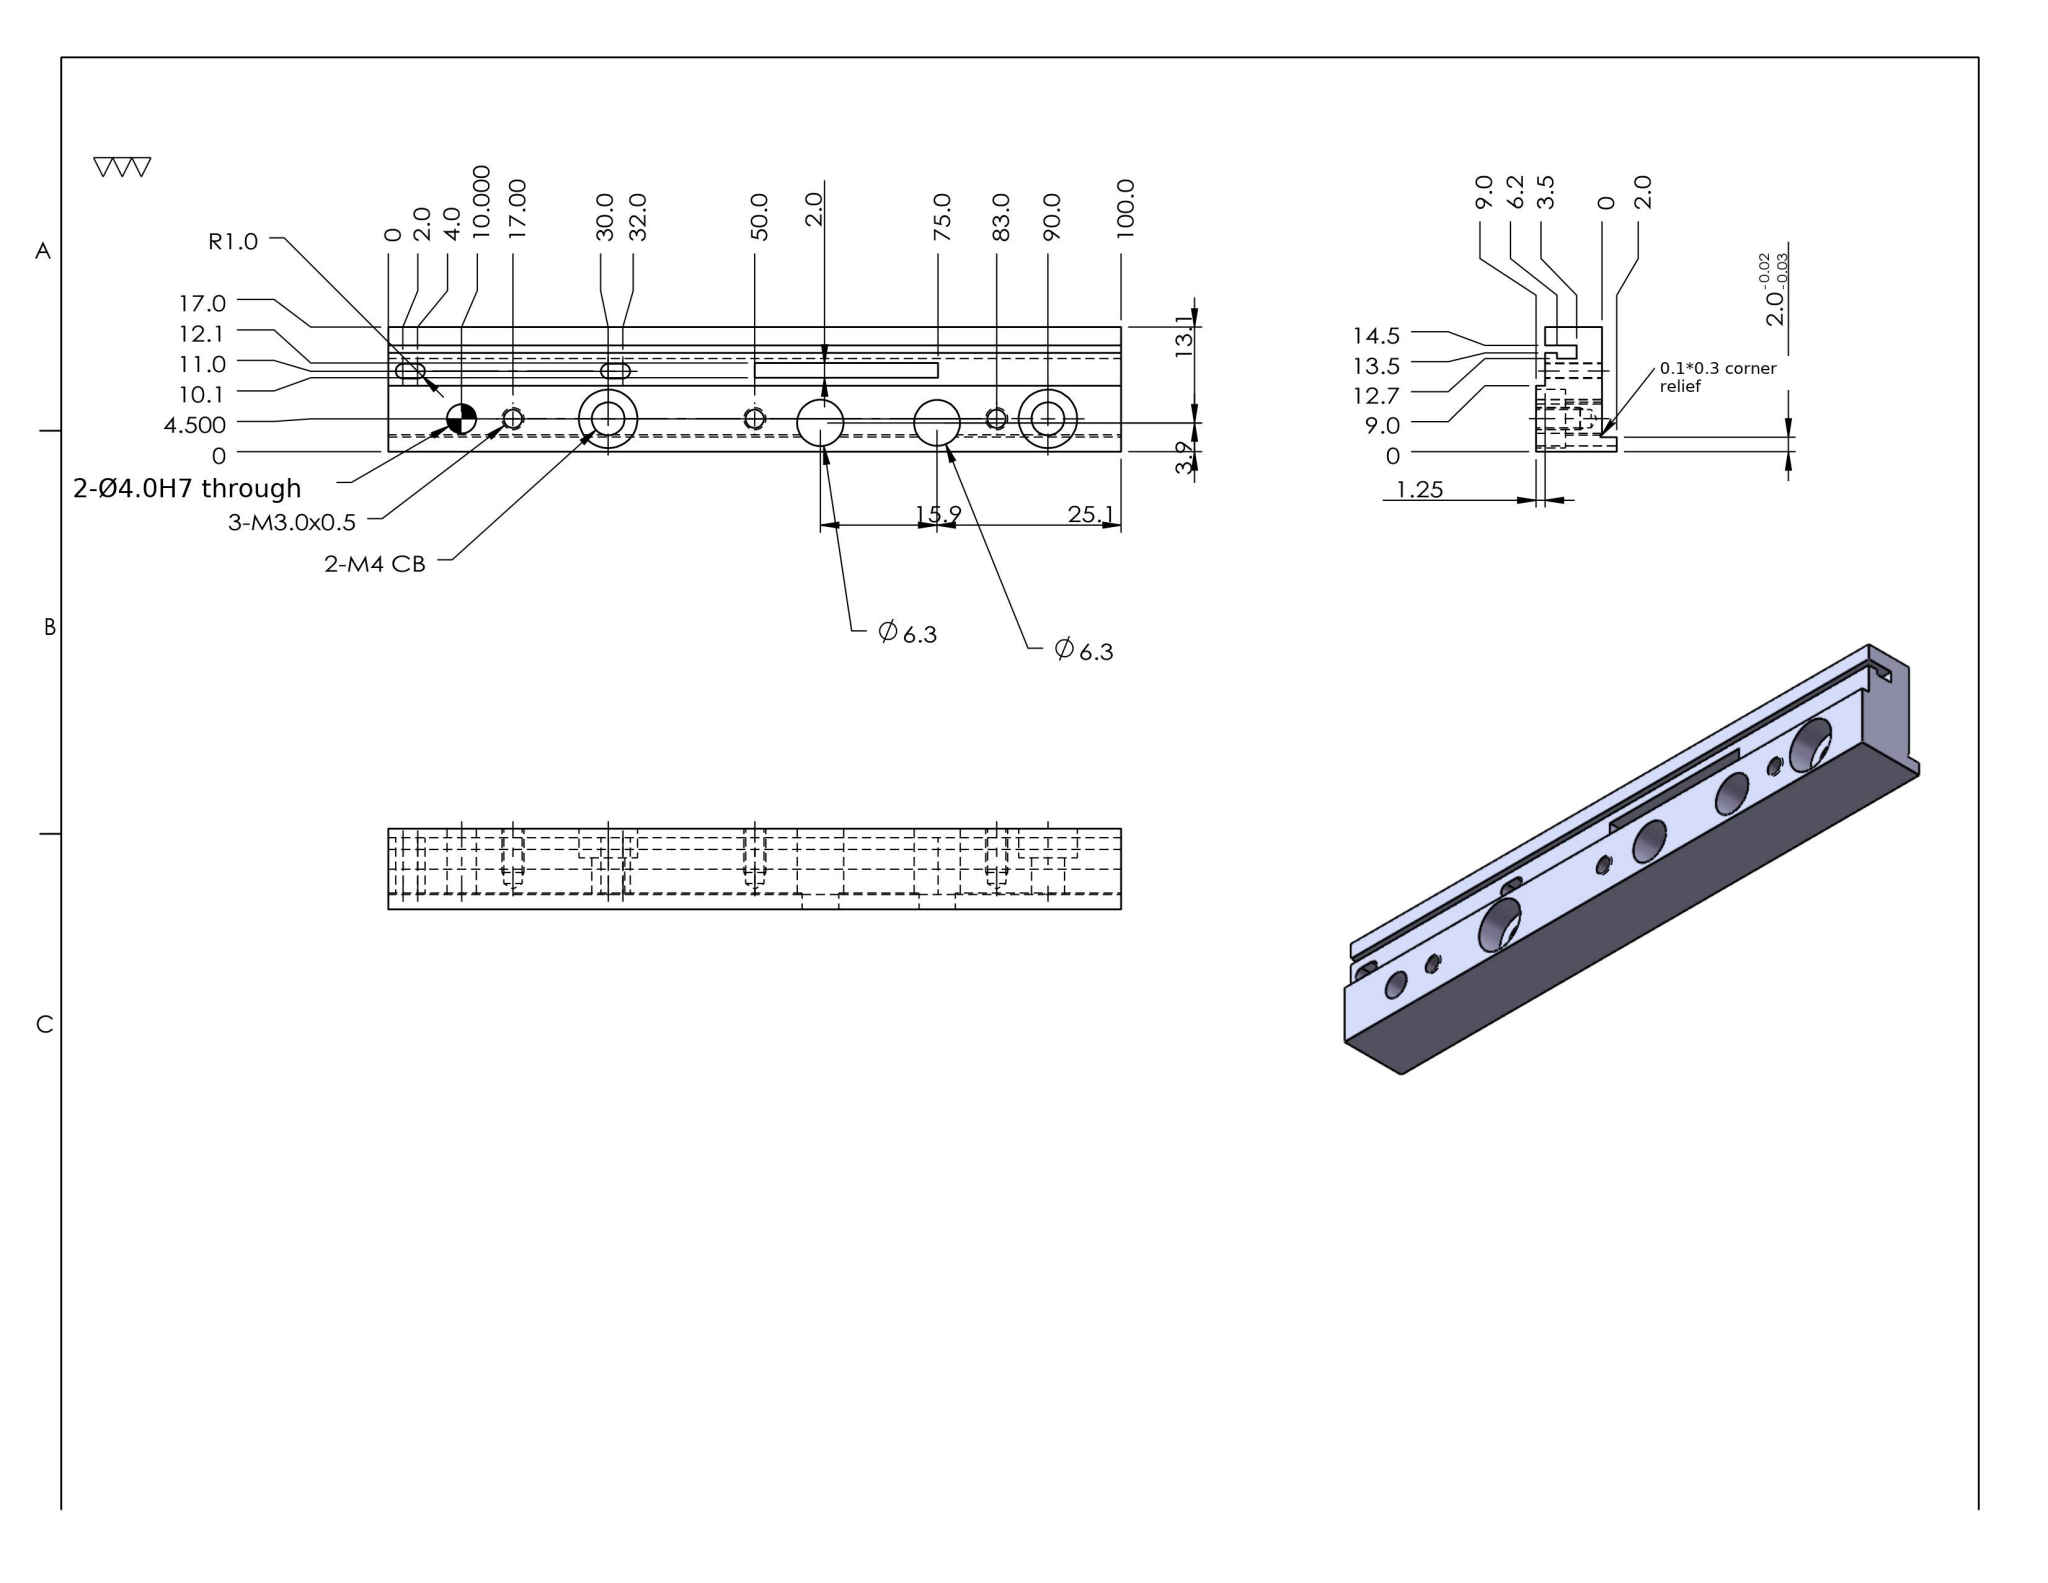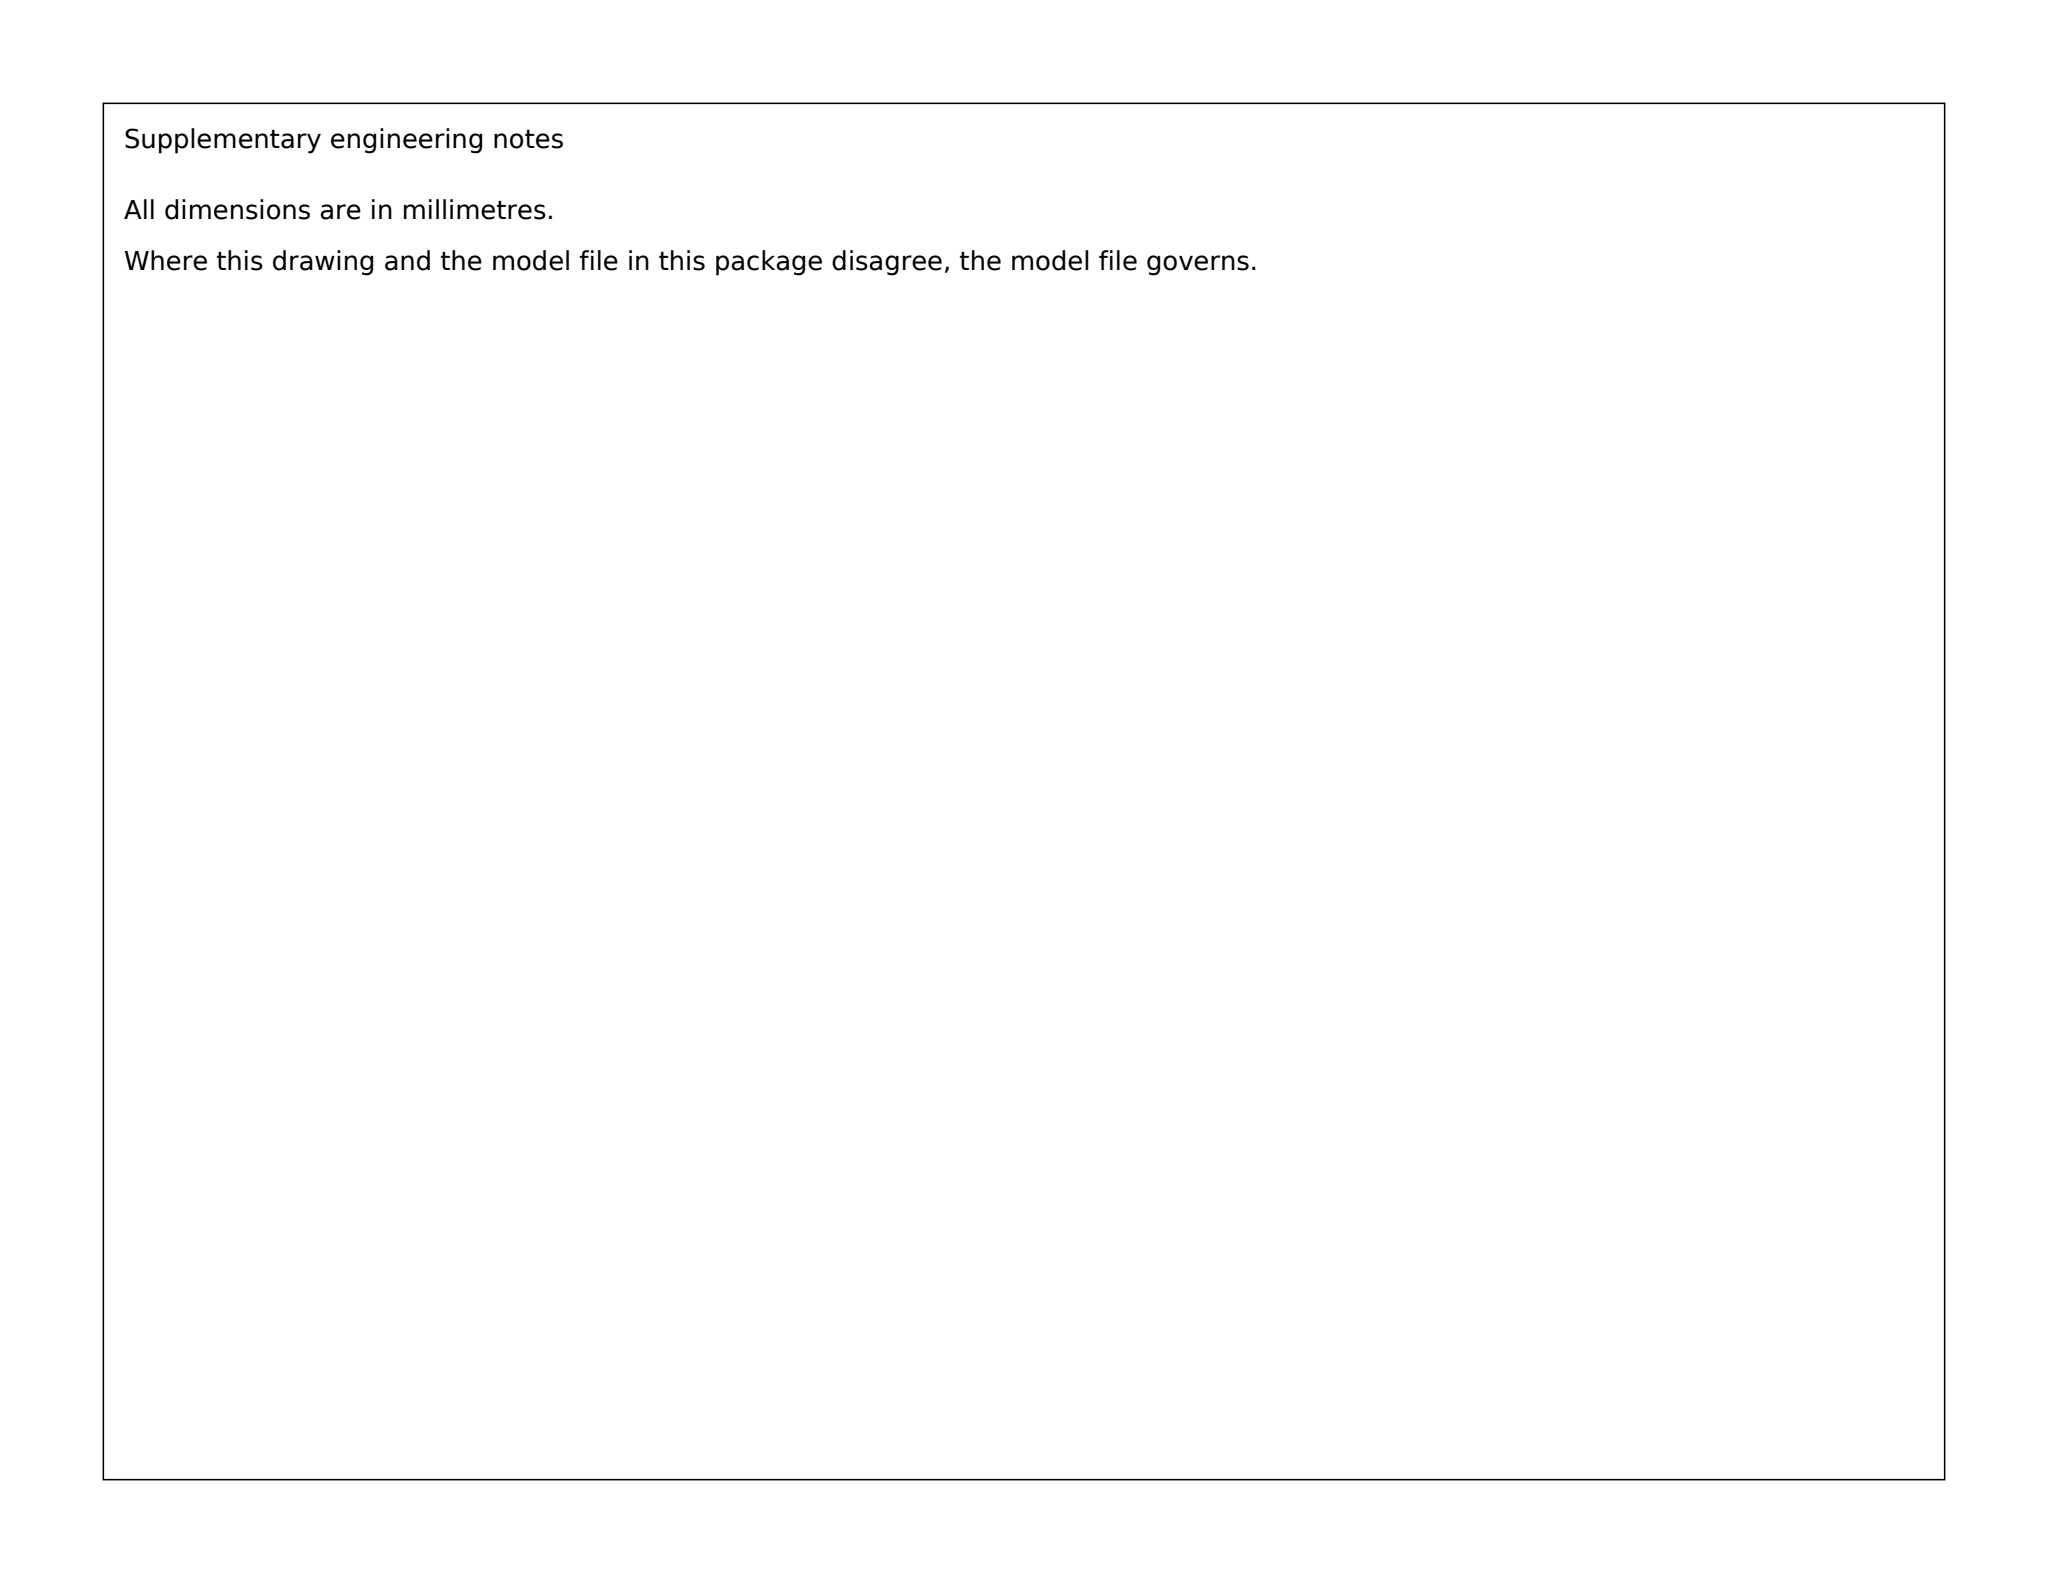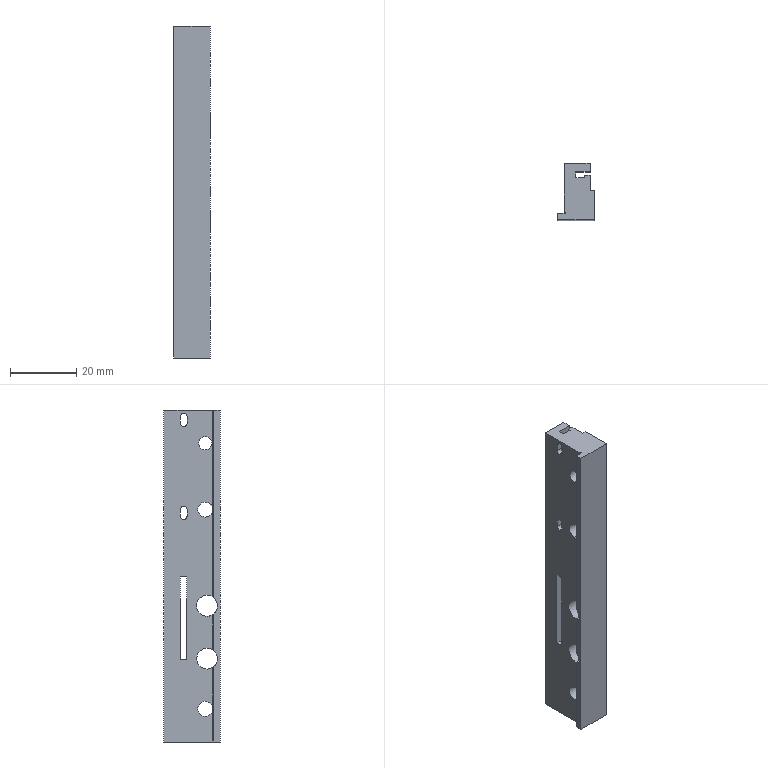Part | SolidWorks | mm | 1 solid | 68 faces | box 11 x 17 x 100 mm | volume 12182 mm3 | plane 36 | cylinder 26 | cone 6 | commonest cylinder face diameters 2.5 x6 2 x6 8 x4 4.5 x4 6.339 x2 6.289 x2 4 x2
build123d program:
from build123d import *

# Parameters (mm, degrees)
SKETCH1_W                                            = 240
SKETCH1_H                                            = 30
EXTRUDE1_DEPTH                                       = 9
SKETCH2_W                                            = 240
SKETCH2_H                                            = 8
EXTRUDE2_DEPTH                                       = 1.25
SKETCH3_W                                            = 4.3
SKETCH3_H                                            = 1
EXTRUDE3_DEPTH                                       = 243.035
SKETCH5_W                                            = 9
SKETCH5_H                                            = 9
CUT_EXTRUDE1_DEPTH                                   = 243.035
CHAMFER1_SIZE                                        = 0.5
CHAMFER1_SIZE2                                       = 3
CHAMFER2_SIZE                                        = 3
CHAMFER2_SIZE2                                       = 0.5
CHAMFER3_SIZE                                        = 0.3
CHAMFER3_SIZE2                                       = 3
CYLINDRICAL_COUNTERSUNK_HOLE_FOR_M4_SOCK_D           = 4.5
CYLINDRICAL_COUNTERSUNK_HOLE_FOR_M4_SOCK_CBORE_D     = 8
CYLINDRICAL_COUNTERSUNK_HOLE_FOR_M4_SOCK_CBORE_DEPTH = 4
LPATTERN1_COUNT                                      = 4
LPATTERN1_PITCH                                      = 60
SKETCH8_W                                            = 2
SKETCH8_H                                            = 2
EXTRUDE5_DEPTH                                       = 240
SKETCH9_W                                            = 0.2
SKETCH9_H                                            = 0.3
EXTRUDE6_DEPTH                                       = 242.085
SKETCH10_W                                           = 9
SKETCH10_H                                           = 4
EXTRUDE7_DEPTH                                       = 242.085
SKETCH11_R                                           = 2
CUT_EXTRUDE2_DEPTH                                   = 241.853
SKETCH12_W                                           = 2.7
SKETCH12_H                                           = 0.8
EXTRUDE8_DEPTH                                       = 241.77
SKETCH13_W                                           = 25
SKETCH13_H                                           = 2
CUT_EXTRUDE3_DEPTH                                   = 241.799
SKETCH15_R                                           = 0.75
CUT_EXTRUDE4_DEPTH                                   = 241.799
EXTRUDE9_DEPTH                                       = 241.799
SKETCH17_W                                           = 15
SKETCH17_H                                           = 9
CUT_EXTRUDE5_DEPTH                                   = 1.2
M3X0_5_TAPPED_HOLE1_D                                = 2.5
M3X0_5_TAPPED_HOLE1_DEPTH                            = 7.5
M3X0_5_TAPPED_HOLE1_TIP                              = 0.7511
SKETCH20_W                                           = 5
SKETCH20_H                                           = 3
CUT_EXTRUDE6_DEPTH                                   = 241.799
FILLET1_R                                            = 0.3
SKETCH21_OUTSIDE_W                                   = 290.17
SKETCH21_OUTSIDE_H                                   = 67.17
SKETCH21_OUTSIDE_W_2                                 = 100
SKETCH21_OUTSIDE_H_2                                 = 17
EXTRUDE10_DEPTH                                      = 241.853
SKETCH22_R                                           = 3.17
SKETCH22_R_2                                         = 3.144
CUT_EXTRUDE7_DEPTH                                   = 42


with BuildPart() as part:
    # Sketch1 → Extrude1 (new body)
    with BuildSketch(Plane(origin=(0, 0, 0), x_dir=(0, 0, -1), z_dir=(1, 0, 0))):
        with Locations((120, 15)):
            Rectangle(SKETCH1_W, SKETCH1_H)
    extrude(amount=EXTRUDE1_DEPTH)

    # Sketch2 → Extrude2 (cut)
    with BuildSketch(Plane(origin=(9, 0, 0), x_dir=(0, 0, -1), z_dir=(1, 0, 0))):
        with Locations((120, 13)):
            Rectangle(SKETCH2_W, SKETCH2_H)
    extrude(amount=-EXTRUDE2_DEPTH, mode=Mode.SUBTRACT)

    # Sketch3 → Extrude3 (cut, through all)
    with BuildSketch(Plane(origin=(0, 0, -240), x_dir=(-1, 0, 0), z_dir=(0, 0, -1))):
        with Locations((-5.6, 14)):
            Rectangle(SKETCH3_W, SKETCH3_H)
    extrude(amount=-EXTRUDE3_DEPTH, mode=Mode.SUBTRACT)

    # Sketch5 → Cut-Extrude1 (cut, through all)
    with BuildSketch(Plane(origin=(0, 0, -240), x_dir=(-1, 0, 0), z_dir=(0, 0, -1))):
        with Locations((-4.5, 25.5)):
            Rectangle(SKETCH5_W, SKETCH5_H)
    extrude(amount=-CUT_EXTRUDE1_DEPTH, mode=Mode.SUBTRACT)

    # Chamfer1
    chamfer1_edges = [part.edges().sort_by_distance(p)[0] for p in [
        (7.75, 11.25, -240),
        (7.75, 15.75, -240),
    ]]
    chamfer1_side = [part.faces().sort_by_distance(p)[0] for p in [
        (4.251, 10.271, -240),
    ]]
    chamfer(chamfer1_edges, length=CHAMFER1_SIZE, length2=CHAMFER1_SIZE2, reference=chamfer1_side[0])

    # Chamfer2
    chamfer2_edges = [part.edges().sort_by_distance(p)[0] for p in [
        (8.125, 9, -240),
    ]]
    chamfer2_side = [part.faces().sort_by_distance(p)[0] for p in [
        (8.373, 9, -120.297),
    ]]
    chamfer(chamfer2_edges, length=CHAMFER2_SIZE, length2=CHAMFER2_SIZE2, reference=chamfer2_side[0])

    # Chamfer3
    chamfer3_edges = [part.edges().sort_by_distance(p)[0] for p in [
        (5.35, 14.5, -240),
        (5.35, 13.5, -240),
    ]]
    chamfer3_side = [part.faces().sort_by_distance(p)[0] for p in [
        (4.164, 10.225, -240),
    ]]
    chamfer(chamfer3_edges, length=CHAMFER3_SIZE, length2=CHAMFER3_SIZE2, reference=chamfer3_side[0])

    # Cylindrical Countersunk Hole for M4 Sock (through all)
    with Locations(Plane(origin=(9, 0, 0), x_dir=(0, 0, -1), z_dir=(1, 0, 0))):
        with Locations((30, 4.5)):
            cylindrical_countersunk_hole_for_m4_sock = CounterBoreHole(CYLINDRICAL_COUNTERSUNK_HOLE_FOR_M4_SOCK_D / 2, CYLINDRICAL_COUNTERSUNK_HOLE_FOR_M4_SOCK_CBORE_D / 2, CYLINDRICAL_COUNTERSUNK_HOLE_FOR_M4_SOCK_CBORE_DEPTH)

    # LPattern1: Cylindrical Countersunk Hole for M4 Sock ×4
    with Locations(*[(0, 0, -i * LPATTERN1_PITCH) for i in range(1, LPATTERN1_COUNT)]):
        add(cylindrical_countersunk_hole_for_m4_sock, mode=Mode.SUBTRACT)

    # Sketch8 → Extrude5 (add)
    with BuildSketch(Plane(origin=(0, 0, -240), x_dir=(-1, 0, 0), z_dir=(0, 0, -1))):
        with Locations((1, 1)):
            Rectangle(SKETCH8_W, SKETCH8_H)
    extrude(amount=-EXTRUDE5_DEPTH)

    # Sketch9 → Extrude6 (cut, through all)
    with BuildSketch(Plane(origin=(0, 0, -240), x_dir=(-1, 0, 0), z_dir=(0, 0, -1))):
        with Locations((-0.1, 2.15)):
            Rectangle(SKETCH9_W, SKETCH9_H)
    extrude(amount=-EXTRUDE6_DEPTH, mode=Mode.SUBTRACT)

    # Sketch10 → Extrude7 (cut, through all)
    with BuildSketch(Plane(origin=(0, 0, -240), x_dir=(-1, 0, 0), z_dir=(0, 0, -1))):
        with Locations((-4.5, 19)):
            Rectangle(SKETCH10_W, SKETCH10_H)
    extrude(amount=-EXTRUDE7_DEPTH, mode=Mode.SUBTRACT)

    # Sketch11 → Cut-Extrude2 (cut, through all)
    with BuildSketch(Plane(origin=(9, 0, 0), x_dir=(0, 0, -1), z_dir=(1, 0, 0))):
        with Locations((10, 4.5)):
            Circle(SKETCH11_R)
    extrude(amount=-CUT_EXTRUDE2_DEPTH, mode=Mode.SUBTRACT)

    # Sketch12 → Extrude8 (cut, through all)
    with BuildSketch(Plane.XY):
        with Locations((4.8, 13.1)):
            Rectangle(SKETCH12_W, SKETCH12_H)
    extrude(amount=-EXTRUDE8_DEPTH, mode=Mode.SUBTRACT)

    # Sketch13 → Cut-Extrude3 (cut, through all)
    with BuildSketch(Plane(origin=(7.75, 0, 0), x_dir=(0, 0, -1), z_dir=(1, 0, 0))):
        with Locations((62.5, 11.1)):
            Rectangle(SKETCH13_W, SKETCH13_H)
    extrude(amount=-CUT_EXTRUDE3_DEPTH, mode=Mode.SUBTRACT)

    # Sketch15 → Cut-Extrude4 (cut, through all)
    with BuildSketch(Plane(origin=(7.75, 0, 0), x_dir=(0, 0, -1), z_dir=(1, 0, 0))):
        with Locations((3, 11)):
            Circle(SKETCH15_R)
        with Locations((31, 11)):
            Circle(SKETCH15_R)
    extrude(amount=-CUT_EXTRUDE4_DEPTH, mode=Mode.SUBTRACT)

    # Sketch16 → Extrude9 (cut, through all)
    with BuildSketch(Plane(origin=(7.75, 0, 0), x_dir=(0, 0, -1), z_dir=(1, 0, 0))):
        with BuildLine():
            Line((2, 12), (4, 12))
            ThreePointArc((4, 12), (5, 11), (4, 10))
            Line((4, 10), (2, 10))
            ThreePointArc((2, 10), (1, 11), (2, 12))
        make_face()
        with BuildLine():
            Line((32, 10), (30, 10))
            ThreePointArc((30, 10), (29, 11), (30, 12))
            Line((30, 12), (32, 12))
            ThreePointArc((32, 12), (33, 11), (32, 10))
        make_face()
    extrude(amount=-EXTRUDE9_DEPTH, mode=Mode.SUBTRACT)

    # Sketch17 → Cut-Extrude5 (cut)
    with BuildSketch(Plane(origin=(9, 0, 0), x_dir=(0, 0, -1), z_dir=(1, 0, 0))):
        with Locations((172.5, 4.5)):
            Rectangle(SKETCH17_W, SKETCH17_H)
    extrude(amount=-CUT_EXTRUDE5_DEPTH, mode=Mode.SUBTRACT)

    # M3x0.5 Tapped Hole1
    with Locations(Plane(origin=(9, 0, 0), x_dir=(0, 0, -1), z_dir=(1, 0, 0))):
        with Locations((230, 4.5), (200, 4.5), (140, 4.5), (110, 4.5), (83, 4.5), (50, 4.5), (17, 4.5)):
            Hole(M3X0_5_TAPPED_HOLE1_D / 2, depth=M3X0_5_TAPPED_HOLE1_DEPTH)
            with Locations((0, 0, -(M3X0_5_TAPPED_HOLE1_DEPTH + M3X0_5_TAPPED_HOLE1_TIP / 2))):  # 118° drill point
                Cone(0, M3X0_5_TAPPED_HOLE1_D / 2, M3X0_5_TAPPED_HOLE1_TIP, mode=Mode.SUBTRACT)

    # Sketch20 → Cut-Extrude6 (cut, through all)
    with BuildSketch(Plane(origin=(7.75, 0, 0), x_dir=(0, 0, -1), z_dir=(1, 0, 0))):
        with Locations((123, 11)):
            Rectangle(SKETCH20_W, SKETCH20_H)
    extrude(amount=-CUT_EXTRUDE6_DEPTH, mode=Mode.SUBTRACT)

    # Fillet1
    fillet1_edges = [part.edges().sort_by_distance(p)[0] for p in [
        (3.875, 12.5, -125.5),
        (3.875, 9.5, -125.5),
        (3.875, 9.5, -120.5),
        (3.875, 12.5, -120.5),
    ]]
    fillet(fillet1_edges, radius=FILLET1_R)

    # Sketch21 outside → Extrude10 (cut, through all)
    with BuildSketch(Plane(origin=(9, 0, 0), x_dir=(0, 0, -1), z_dir=(1, 0, 0))):
        with Locations((120, 8.5)):
            Rectangle(SKETCH21_OUTSIDE_W, SKETCH21_OUTSIDE_H)
        with Locations((50, 8.5)):
            Rectangle(SKETCH21_OUTSIDE_W_2, SKETCH21_OUTSIDE_H_2, mode=Mode.SUBTRACT)
    extrude(amount=-EXTRUDE10_DEPTH, mode=Mode.SUBTRACT)

    # Sketch22 → Cut-Extrude7 (cut)
    with BuildSketch(Plane(origin=(9, 0, 0), x_dir=(0, 0, -1), z_dir=(1, 0, 0))):
        with Locations((58.949, 3.943)):
            Circle(SKETCH22_R)
        with Locations((74.879, 3.943)):
            Circle(SKETCH22_R_2)
    extrude(amount=-CUT_EXTRUDE7_DEPTH, mode=Mode.SUBTRACT)


solid = part.part